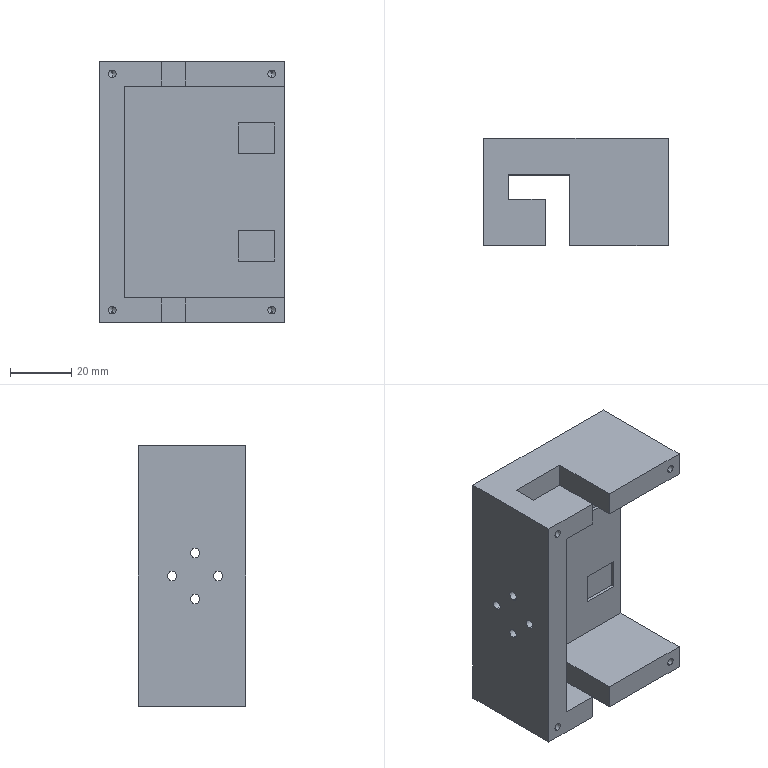Component | SolidWorks | WheelAssembly-1_Bracket-1 | 1 solid | 59 faces | box 60 x 35 x 85 mm | volume 75334 mm3 | plane 33 | cylinder 18 | cone 8 | commonest cylinder face diameters 3 x8 2.5 x8 20 x2
build123d program:
from build123d import *

# Parameters (mm, degrees)
SKETCH1_2_W           = 35
SKETCH1_2_H           = 60
BOSS_EXTRUDE1_DEPTH   = 42.5
SHELL1_T              = -8
CUT_EXTRUDE1_2_DEPTH  = 100
M3_TAPPED_HOLE1_D     = 2.5
M3_TAPPED_HOLE1_DEPTH = 7.5
M3_TAPPED_HOLE1_TIP   = 0.7511
SKETCH5_R             = 10
CUT_EXTRUDE2_DEPTH    = 4
SKETCH6_R             = 1.5
CUT_EXTRUDE3_DEPTH    = 73.447
SKETCH1_W             = 10
SKETCH1_H             = 12
CUT_EXTRUDE1_DEPTH    = 1.2


with BuildPart() as part:
    # Sketch1_2 → Boss-Extrude1 (new, symmetric)
    with BuildSketch(Plane.XY):
        Rectangle(SKETCH1_2_W, SKETCH1_2_H)
    extrude(amount=BOSS_EXTRUDE1_DEPTH, both=True)

    # Shell1
    shell1_openings = [part.faces().sort_by_distance(p)[0] for p in [
        (0, -30, 0),
        (17.5, 0, 0),
    ]]
    offset(amount=SHELL1_T, openings=shell1_openings, kind=Kind.INTERSECTION)

    # Sketch2 → Cut-Extrude1_2 (cut)
    with BuildSketch(Plane.XY.offset(42.5)):
        Polygon((-5.5, 22), (-5.5, 2), (17.5, 2), (17.5, 10), (2.5, 10), (2.5, 22), align=None)
    extrude(amount=-CUT_EXTRUDE1_2_DEPTH, mode=Mode.SUBTRACT)

    # M3 Tapped Hole1
    with Locations(Plane(origin=(17.5, 0, 0), x_dir=(0, 0, -1), z_dir=(1, 0, 0))):
        with Locations((-38.5, 26), (38.5, 26), (38.5, -26), (-38.5, -26)):
            Hole(M3_TAPPED_HOLE1_D / 2, depth=M3_TAPPED_HOLE1_DEPTH)
            with Locations((0, 0, -(M3_TAPPED_HOLE1_DEPTH + M3_TAPPED_HOLE1_TIP / 2))):  # 118° drill point
                Cone(0, M3_TAPPED_HOLE1_D / 2, M3_TAPPED_HOLE1_TIP, mode=Mode.SUBTRACT)

    # Sketch5 → Cut-Extrude2 (cut)
    with BuildSketch(Plane.XZ.offset(-22)):
        with Locations(Location((1, 0, 0), (0, 0, 270))):
            Circle(SKETCH5_R)
    extrude(amount=-CUT_EXTRUDE2_DEPTH, mode=Mode.SUBTRACT)

    # Sketch6 → Cut-Extrude3 (cut, through all)
    with BuildSketch(Plane.XZ.offset(-26)):
        with Locations(Location((8.5, 0, 0), (0, 0, 270))):
            Circle(SKETCH6_R)
        with Locations(Location((1, -7.5, 0), (0, 0, 270))):
            Circle(SKETCH6_R)
        with Locations(Location((-6.5, 0, 0), (0, 0, 270))):
            Circle(SKETCH6_R)
        with Locations(Location((1, 7.5, 0), (0, 0, 270))):
            Circle(SKETCH6_R)
    extrude(amount=-CUT_EXTRUDE3_DEPTH, mode=Mode.SUBTRACT)

    # Sketch1 → Cut-Extrude1 (cut)
    with BuildSketch(Plane(origin=(-9.5, 0, 0), x_dir=(0, 0, -1), z_dir=(1, 0, 0))):
        with Locations((-17.5, -21)):
            Rectangle(SKETCH1_W, SKETCH1_H)
        with Locations((17.5, -21)):
            Rectangle(SKETCH1_W, SKETCH1_H)
    extrude(amount=-CUT_EXTRUDE1_DEPTH, mode=Mode.SUBTRACT)


solid = part.part

# Placed as in the assembly
solid = solid.moved(Location((-350, -130.5, -542.97), (180, 0, 90)))